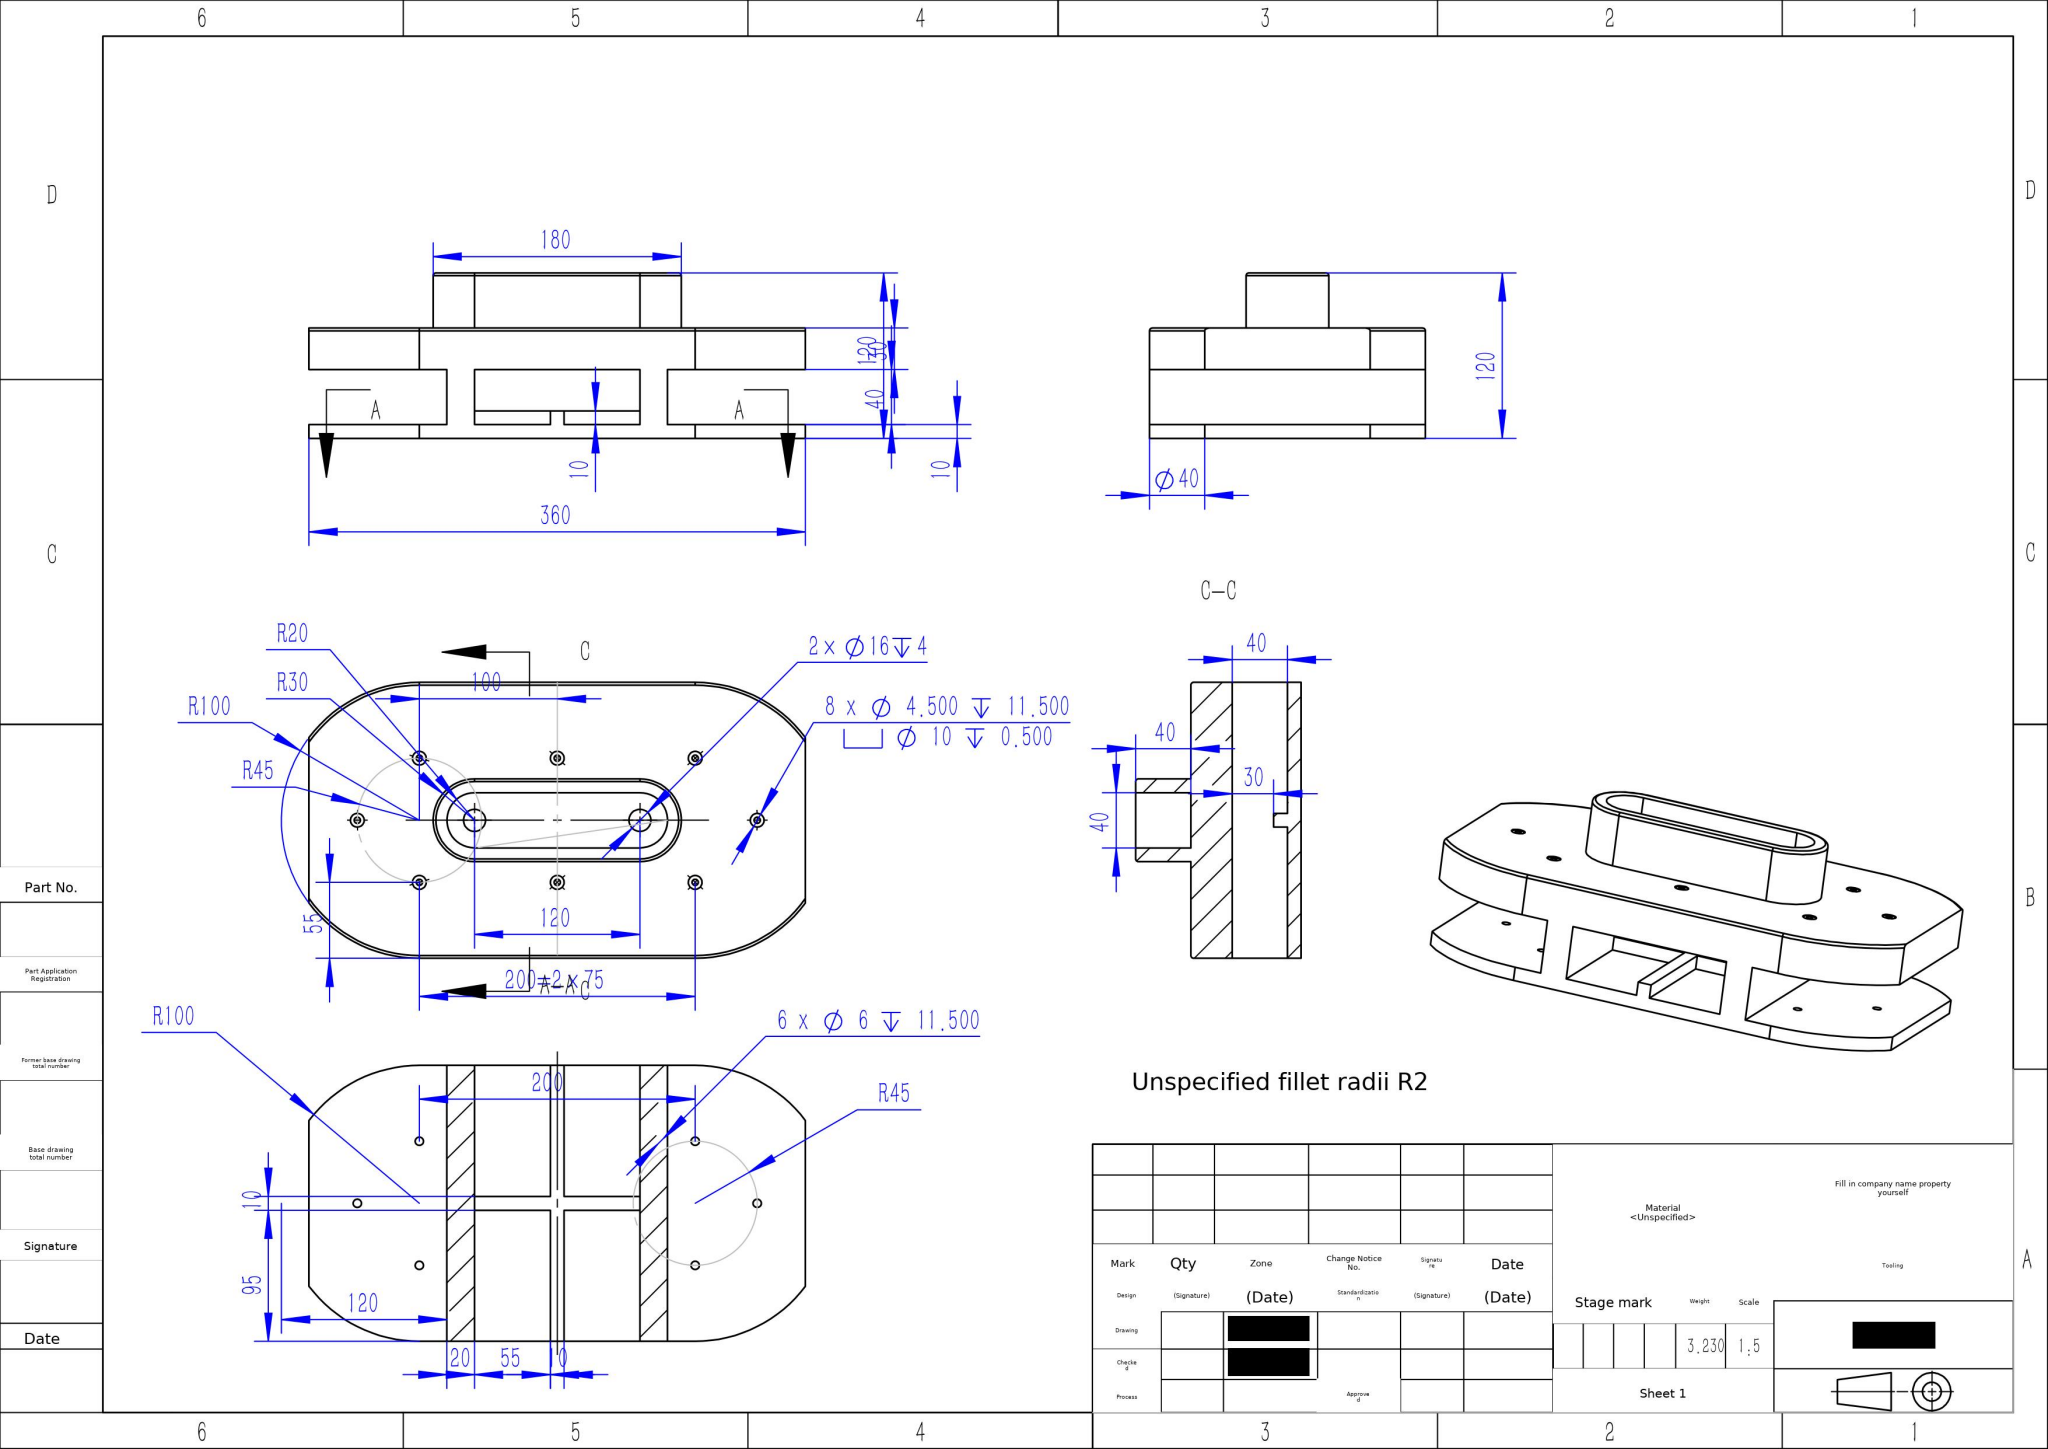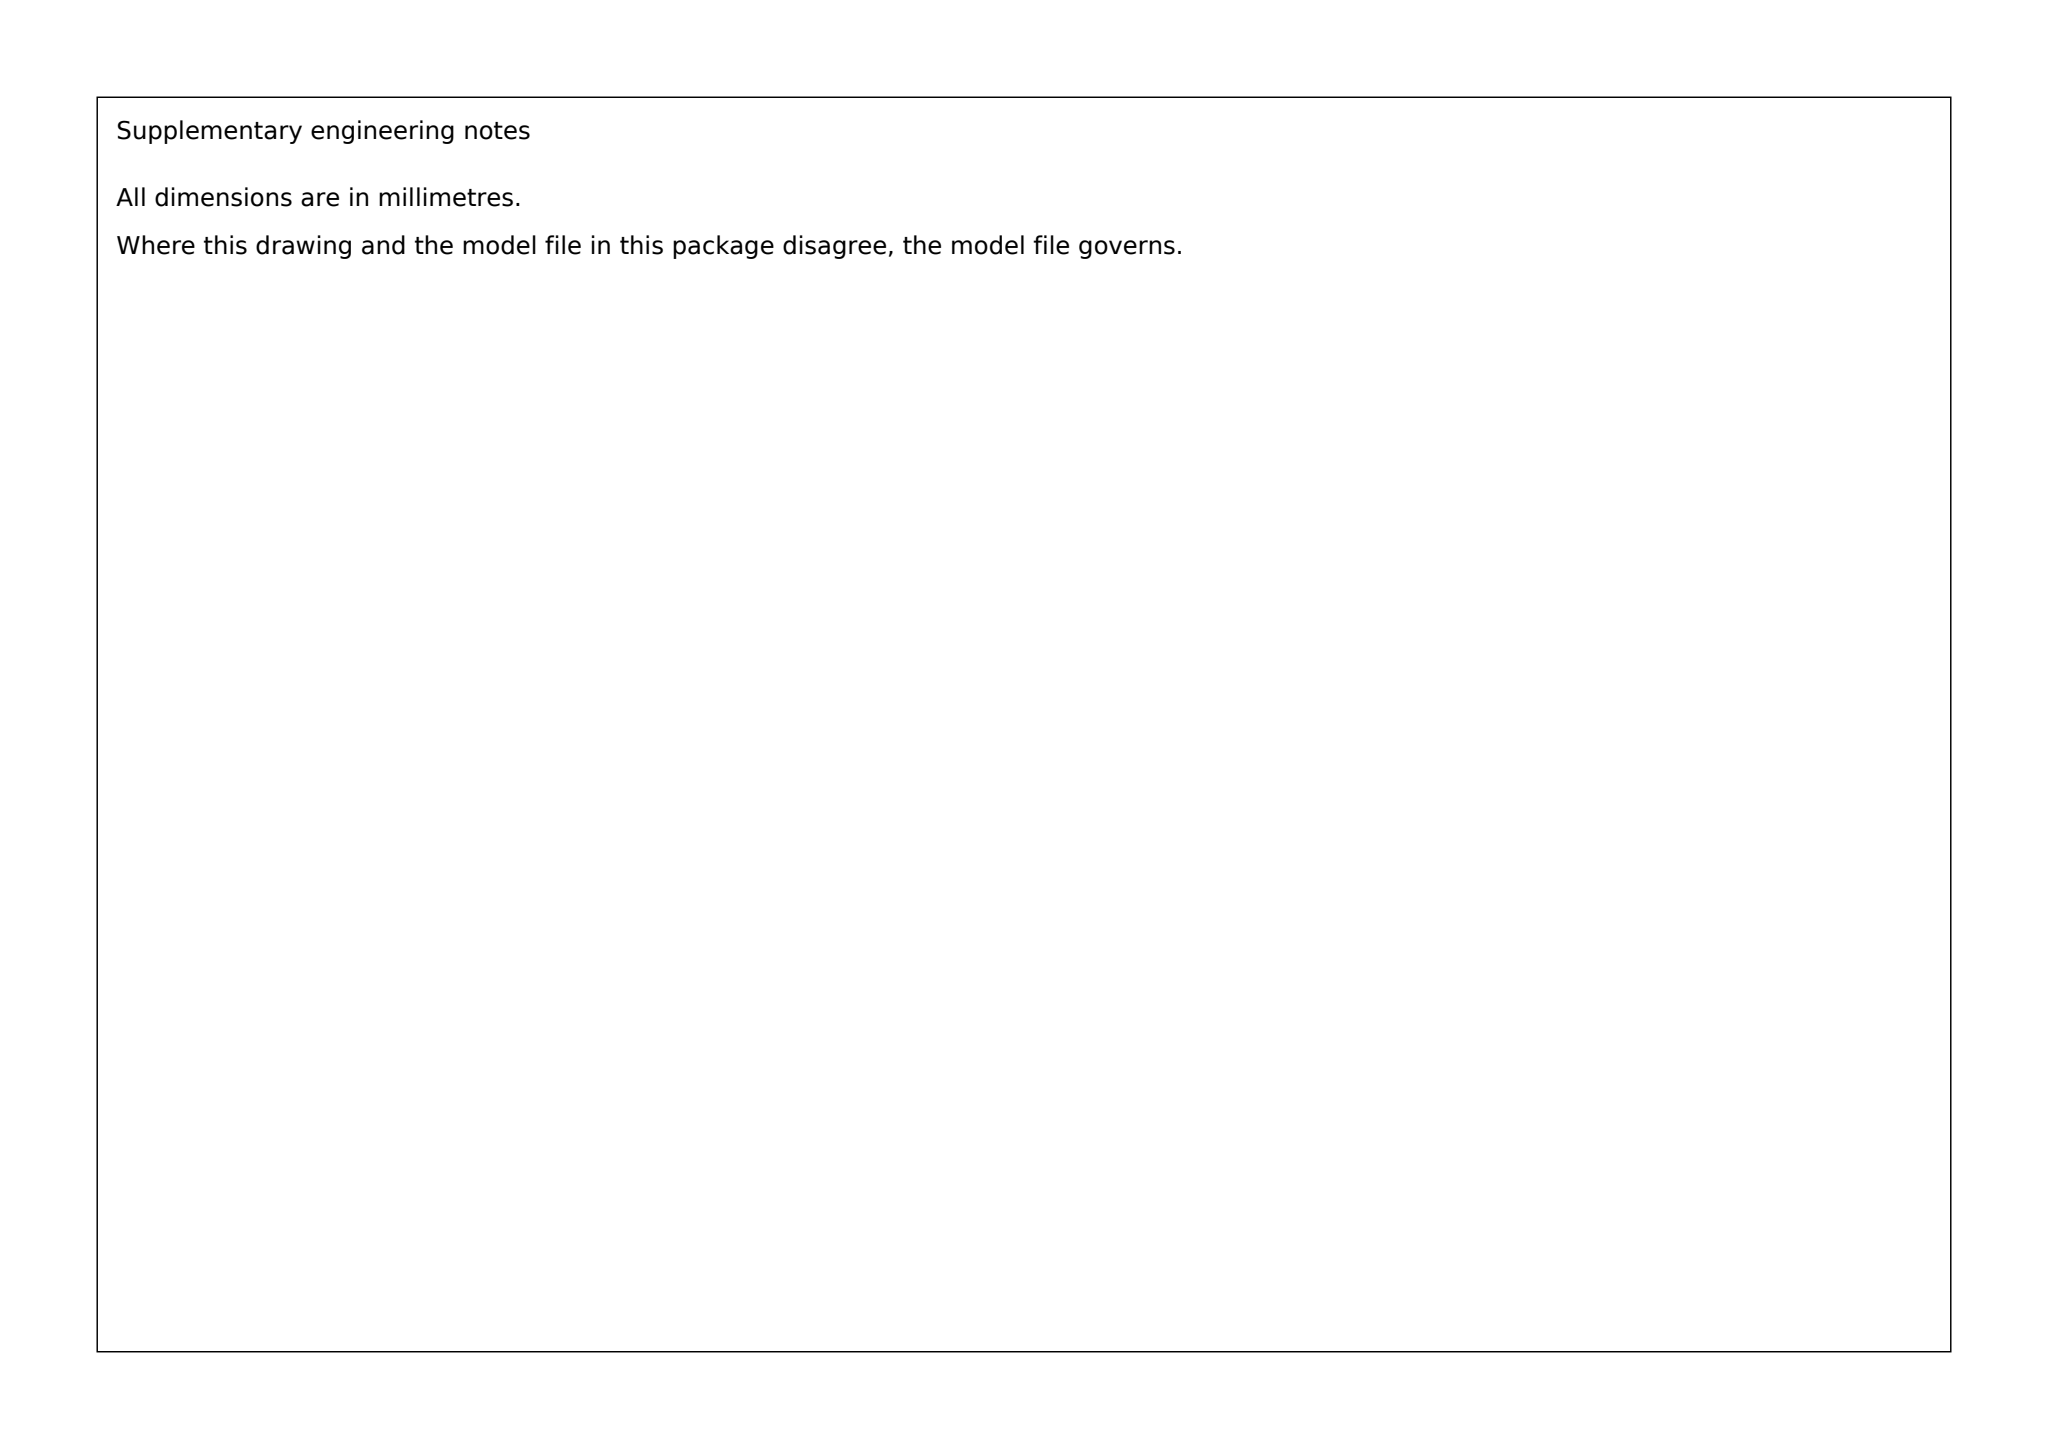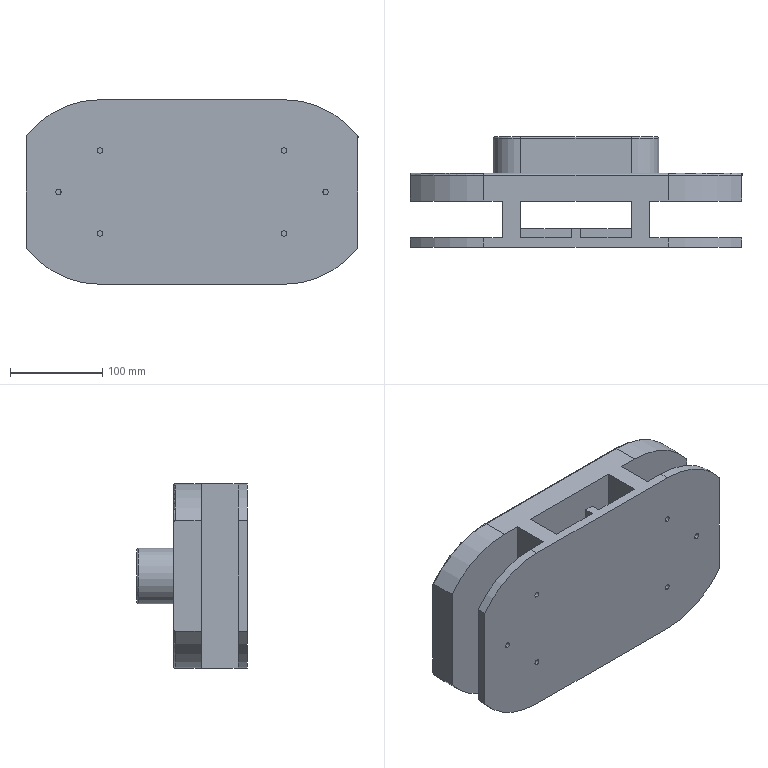Part | SolidWorks | mm | 1 solid | 132 faces | box 360 x 120 x 200 mm | volume 3229564 mm3 | cylinder 64 | plane 46 | cone 16 | torus 6 | commonest cylinder face diameters 10 x16 4.5 x16 6 x12 200 x8 16 x4 4 x4 60 x2 40 x2
build123d program:
from build123d import *

# Parameters (mm, degrees)
BOSS_EXTRUDE1_DEPTH                                 = 10
SKETCH2_W                                           = 20
SKETCH2_H                                           = 200
BOSS_EXTRUDE2_DEPTH                                 = 40
BOSS_EXTRUDE3_DEPTH                                 = 30
BOSS_EXTRUDE4_DEPTH                                 = 40
BOSS_EXTRUDE5_DEPTH                                 = 10
CYLINDRICAL_COUNTERSUNK_HOLE_FOR_M4_HEX_D           = 4.5
CYLINDRICAL_COUNTERSUNK_HOLE_FOR_M4_HEX_DEPTH       = 11.5
CYLINDRICAL_COUNTERSUNK_HOLE_FOR_M4_HEX_CBORE_D     = 10
CYLINDRICAL_COUNTERSUNK_HOLE_FOR_M4_HEX_CBORE_DEPTH = 0.5
CYLINDRICAL_COUNTERSUNK_HOLE_FOR_M4_HEX_TIP         = 1.352
F_6_0_6_DIAMETER_HOLE1_D                            = 6
F_6_0_6_DIAMETER_HOLE1_DEPTH                        = 11.5
F_6_0_6_DIAMETER_HOLE1_TIP                          = 1.803
FILLET1_R                                           = 2
CUT_EXTRUDE2_DEPTH                                  = 40
SKETCH12_R                                          = 8
CUT_EXTRUDE1_DEPTH                                  = 4
SKETCH14_W                                          = 35.635
SKETCH14_H                                          = 256.299
CUT_EXTRUDE3_DEPTH                                  = 238.487


with BuildPart() as part:
    # Sketch1 → Boss-Extrude1 (new body)
    with BuildSketch(Plane(origin=(0, 0, 0), x_dir=(1, 0, 0), z_dir=(0, 1, 0))):
        with BuildLine():
            Line((-100, 100), (100, 100))
            ThreePointArc((100, 100), (200, 0), (100, -100))
            Line((100, -100), (-100, -100))
            ThreePointArc((-100, -100), (-200, 0), (-100, 100))
        make_face()
    extrude(amount=BOSS_EXTRUDE1_DEPTH)

    # Sketch2 → Boss-Extrude2 (add)
    with BuildSketch(Plane(origin=(0, 10, 0), x_dir=(1, 0, 0), z_dir=(0, 1, 0))):
        with Locations((-70, 0)):
            Rectangle(SKETCH2_W, SKETCH2_H)
        with Locations((70, 0)):
            Rectangle(SKETCH2_W, SKETCH2_H)
    extrude(amount=BOSS_EXTRUDE2_DEPTH)

    # Sketch3 → Boss-Extrude3 (add)
    with BuildSketch(Plane(origin=(0, 50, 0), x_dir=(1, 0, 0), z_dir=(0, 1, 0))):
        with BuildLine():
            Line((-100, -100), (-80, -100))
            Line((-80, -100), (-60, -100))
            Line((-60, -100), (60, -100))
            Line((60, -100), (80, -100))
            Line((80, -100), (100, -100))
            ThreePointArc((100, -100), (200, 0), (100, 100))
            Line((100, 100), (80, 100))
            Line((80, 100), (60, 100))
            Line((60, 100), (-60, 100))
            Line((-60, 100), (-80, 100))
            Line((-80, 100), (-100, 100))
            ThreePointArc((-100, 100), (-200, 0), (-100, -100))
        make_face()
    extrude(amount=BOSS_EXTRUDE3_DEPTH)

    # Sketch4 → Boss-Extrude4 (add)
    with BuildSketch(Plane(origin=(0, 80, 0), x_dir=(1, 0, 0), z_dir=(0, 1, 0))):
        with BuildLine():
            Line((-60, 30), (60, 30))
            ThreePointArc((60, 30), (90, 0), (60, -30))
            Line((60, -30), (-60, -30))
            ThreePointArc((-60, -30), (-90, 0), (-60, 30))
        make_face()
    extrude(amount=BOSS_EXTRUDE4_DEPTH)

    # Sketch5 → Boss-Extrude5 (add)
    with BuildSketch(Plane(origin=(0, 10, 0), x_dir=(1, 0, 0), z_dir=(0, 1, 0))):
        Polygon((-60, 5), (-5, 5), (-5, 100), (5, 100), (5, 5), (60, 5), (60, -5), (5, -5), (5, -100), (-5, -100), (-5, -5), (-60, -5), align=None)
    extrude(amount=BOSS_EXTRUDE5_DEPTH)

    # Cylindrical Countersunk Hole for M4 Hex
    with Locations(Plane(origin=(0, 80, 0), x_dir=(1, 0, 0), z_dir=(0, 1, 0))):
        with Locations((-100, 45), (-145, 0), (-100, -45), (100, -45), (145, 0), (100, 45), (0, 45), (0, -45)):
            CounterBoreHole(CYLINDRICAL_COUNTERSUNK_HOLE_FOR_M4_HEX_D / 2, CYLINDRICAL_COUNTERSUNK_HOLE_FOR_M4_HEX_CBORE_D / 2, CYLINDRICAL_COUNTERSUNK_HOLE_FOR_M4_HEX_CBORE_DEPTH, depth=CYLINDRICAL_COUNTERSUNK_HOLE_FOR_M4_HEX_DEPTH)
            with Locations((0, 0, -(CYLINDRICAL_COUNTERSUNK_HOLE_FOR_M4_HEX_DEPTH + CYLINDRICAL_COUNTERSUNK_HOLE_FOR_M4_HEX_TIP / 2))):  # 118° drill point
                Cone(0, CYLINDRICAL_COUNTERSUNK_HOLE_FOR_M4_HEX_D / 2, CYLINDRICAL_COUNTERSUNK_HOLE_FOR_M4_HEX_TIP, mode=Mode.SUBTRACT)

    # 6.0 _6_ Diameter Hole1
    with Locations(Plane(origin=(0, 10, 0), x_dir=(1, 0, 0), z_dir=(0, 1, 0))):
        with Locations((-145, 0), (-100, -45), (100, -45), (145, 0), (100, 45), (-100, 45)):
            Hole(F_6_0_6_DIAMETER_HOLE1_D / 2, depth=F_6_0_6_DIAMETER_HOLE1_DEPTH)
            with Locations((0, 0, -(F_6_0_6_DIAMETER_HOLE1_DEPTH + F_6_0_6_DIAMETER_HOLE1_TIP / 2))):  # 118° drill point
                Cone(0, F_6_0_6_DIAMETER_HOLE1_D / 2, F_6_0_6_DIAMETER_HOLE1_TIP, mode=Mode.SUBTRACT)

    # Fillet1
    fillet1_edges = [part.edges().sort_by_distance(p)[0] for p in [
        (-200, 80, 0),
        (0, 80, 100),
        (200, 80, 0),
        (0, 80, -100),
        (-90, 120, 0),
        (0, 120, 30),
        (90, 120, 0),
        (0, 120, -30),
    ]]
    fillet(fillet1_edges, radius=FILLET1_R)

    # Sketch13 → Cut-Extrude2 (cut)
    with BuildSketch(Plane(origin=(0, 120, 0), x_dir=(1, 0, 0), z_dir=(0, 1, 0))):
        with BuildLine():
            Line((-60, -20), (60, -20))
            ThreePointArc((60, -20), (80, 0), (60, 20))
            Line((60, 20), (-60, 20))
            ThreePointArc((-60, 20), (-80, 0), (-60, -20))
        make_face()
    extrude(amount=-CUT_EXTRUDE2_DEPTH, mode=Mode.SUBTRACT)

    # Sketch12 → Cut-Extrude1 (cut)
    with BuildSketch(Plane(origin=(0, 80, 0), x_dir=(1, 0, 0), z_dir=(0, 1, 0))):
        with Locations(Location((-60, 0, 0), (0, 0, 270))):
            Circle(SKETCH12_R)
        with Locations(Location((60, 0, 0), (0, 0, 270))):
            Circle(SKETCH12_R)
    extrude(amount=-CUT_EXTRUDE1_DEPTH, mode=Mode.SUBTRACT)

    # Sketch14 → Cut-Extrude3 (cut, through all)
    with BuildSketch(Plane(origin=(0, 80, 0), x_dir=(1, 0, 0), z_dir=(0, 1, 0))):
        with Locations((-197.818, 6.673)):
            Rectangle(SKETCH14_W, SKETCH14_H)
        with Locations((197.818, 6.673)):
            Rectangle(SKETCH14_W, SKETCH14_H)
    extrude(amount=-CUT_EXTRUDE3_DEPTH, mode=Mode.SUBTRACT)


solid = part.part